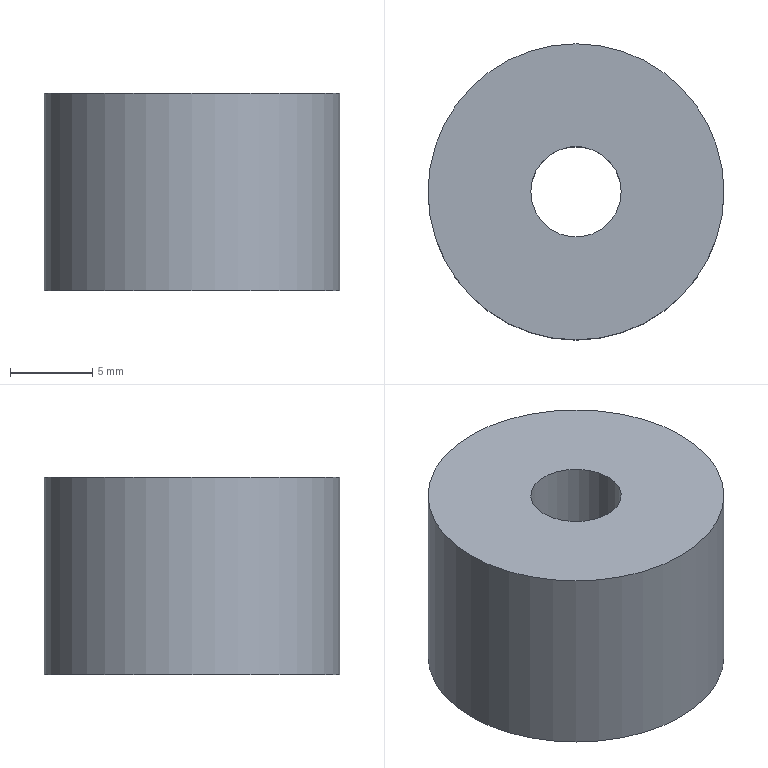Component | NX | BASE_LOC_BLOCK | 1 solid | 6 faces | box 18 x 18 x 12 mm | volume 2473 mm3 | plane 3 | cylinder 3 | commonest cylinder face diameters 18 x1 5.5 x1 10 x1
STEP:
#1=CARTESIAN_POINT('',(0.,0.,0.));
#2=DIRECTION('',(0.,0.,1.));
#3=DIRECTION('',(1.,0.,0.));
#4=AXIS2_PLACEMENT_3D('',#1,#2,#3);
#5=CARTESIAN_POINT('',(110.,0.,-272.));
#6=VERTEX_POINT('',#5);
#7=CARTESIAN_POINT('',(115.,0.,-272.));
#8=DIRECTION('',(0.,0.,1.));
#9=DIRECTION('',(-1.,0.,0.));
#10=AXIS2_PLACEMENT_3D('',#7,#8,#9);
#11=CIRCLE('',#10,5.);
#12=CARTESIAN_POINT('',(115.,0.,-272.));
#13=DIRECTION('',(0.,0.,-1.));
#14=DIRECTION('',(1.,0.,0.));
#15=AXIS2_PLACEMENT_3D('',#12,#13,#14);
#16=PLANE('',#15);
#17=CARTESIAN_POINT('',(-5.,0.));
#18=CARTESIAN_POINT('',(-5.,8.66));
#19=CARTESIAN_POINT('',(2.5,4.33));
#20=CARTESIAN_POINT('',(10.,0.));
#21=CARTESIAN_POINT('',(2.5,-4.33));
#22=CARTESIAN_POINT('',(-5.,-8.66));
#23=CARTESIAN_POINT('',(-5.,0.));
#24=(BOUNDED_CURVE()B_SPLINE_CURVE(2,(#17,#18,#19,#20,#21,#22,#23),.UNSPECIFIED.,.T.,.F.)B_SPLINE_CURVE_WITH_KNOTS((1,2,2,2,2,1),(-2.094,0.,2.094,4.189,6.283,8.378),.UNSPECIFIED.)CURVE()GEOMETRIC_REPRESENTATION_ITEM()RATIONAL_B_SPLINE_CURVE((1.,0.5,1.,0.5,1.,0.5,1.))REPRESENTATION_ITEM(''));
#25=(GEOMETRIC_REPRESENTATION_CONTEXT(2)PARAMETRIC_REPRESENTATION_CONTEXT()REPRESENTATION_CONTEXT('',''));
#26=DEFINITIONAL_REPRESENTATION('',(#24),#25);
#27=PCURVE('',#16,#26);
#28=CARTESIAN_POINT('',(115.,0.,-272.));
#29=DIRECTION('',(0.,0.,1.));
#30=DIRECTION('',(-1.,0.,0.));
#31=AXIS2_PLACEMENT_3D('',#28,#29,#30);
#32=CYLINDRICAL_SURFACE('',#31,5.);
#33=CARTESIAN_POINT('',(0.,0.));
#34=DIRECTION('',(1.,0.));
#35=VECTOR('',#34,1.);
#36=LINE('',#33,#35);
#37=(GEOMETRIC_REPRESENTATION_CONTEXT(2)PARAMETRIC_REPRESENTATION_CONTEXT()REPRESENTATION_CONTEXT('',''));
#38=DEFINITIONAL_REPRESENTATION('',(#36),#37);
#39=PCURVE('',#32,#38);
#40=SURFACE_CURVE('',#11,(#27,#39),.PCURVE_S1.);
#41=EDGE_CURVE('',#6,#6,#40,.T.);
#42=ORIENTED_EDGE('',*,*,#41,.T.);
#43=EDGE_LOOP('',(#42));
#44=FACE_BOUND('',#43,.T.);
#45=CARTESIAN_POINT('',(124.,0.,-272.));
#46=VERTEX_POINT('',#45);
#47=CARTESIAN_POINT('',(115.,0.,-272.));
#48=DIRECTION('',(0.,0.,1.));
#49=DIRECTION('',(1.,0.,0.));
#50=AXIS2_PLACEMENT_3D('',#47,#48,#49);
#51=CIRCLE('',#50,9.);
#52=CARTESIAN_POINT('',(9.,0.));
#53=CARTESIAN_POINT('',(9.,-15.588));
#54=CARTESIAN_POINT('',(-4.5,-7.794));
#55=CARTESIAN_POINT('',(-18.,-0.));
#56=CARTESIAN_POINT('',(-4.5,7.794));
#57=CARTESIAN_POINT('',(9.,15.588));
#58=CARTESIAN_POINT('',(9.,0.));
#59=(BOUNDED_CURVE()B_SPLINE_CURVE(2,(#52,#53,#54,#55,#56,#57,#58),.UNSPECIFIED.,.T.,.F.)B_SPLINE_CURVE_WITH_KNOTS((1,2,2,2,2,1),(-2.094,0.,2.094,4.189,6.283,8.378),.UNSPECIFIED.)CURVE()GEOMETRIC_REPRESENTATION_ITEM()RATIONAL_B_SPLINE_CURVE((1.,0.5,1.,0.5,1.,0.5,1.))REPRESENTATION_ITEM(''));
#60=(GEOMETRIC_REPRESENTATION_CONTEXT(2)PARAMETRIC_REPRESENTATION_CONTEXT()REPRESENTATION_CONTEXT('',''));
#61=DEFINITIONAL_REPRESENTATION('',(#59),#60);
#62=PCURVE('',#16,#61);
#63=CARTESIAN_POINT('',(115.,0.,-260.));
#64=DIRECTION('',(0.,0.,-1.));
#65=DIRECTION('',(1.,0.,0.));
#66=AXIS2_PLACEMENT_3D('',#63,#64,#65);
#67=CYLINDRICAL_SURFACE('',#66,9.);
#68=CARTESIAN_POINT('',(6.283,12.));
#69=DIRECTION('',(-1.,0.));
#70=VECTOR('',#69,1.);
#71=LINE('',#68,#70);
#72=(GEOMETRIC_REPRESENTATION_CONTEXT(2)PARAMETRIC_REPRESENTATION_CONTEXT()REPRESENTATION_CONTEXT('',''));
#73=DEFINITIONAL_REPRESENTATION('',(#71),#72);
#74=PCURVE('',#67,#73);
#75=SURFACE_CURVE('',#51,(#62,#74),.PCURVE_S1.);
#76=EDGE_CURVE('',#46,#46,#75,.T.);
#77=ORIENTED_EDGE('',*,*,#76,.F.);
#78=EDGE_LOOP('',(#77));
#79=FACE_BOUND('',#78,.T.);
#80=ADVANCED_FACE('',(#44,#79),#16,.T.);
#81=CARTESIAN_POINT('',(112.25,0.,-260.));
#82=VERTEX_POINT('',#81);
#83=CARTESIAN_POINT('',(115.,0.,-260.));
#84=DIRECTION('',(0.,0.,1.));
#85=DIRECTION('',(-1.,0.,0.));
#86=AXIS2_PLACEMENT_3D('',#83,#84,#85);
#87=CIRCLE('',#86,2.75);
#88=CARTESIAN_POINT('',(115.,0.,-260.));
#89=DIRECTION('',(0.,0.,1.));
#90=DIRECTION('',(-1.,0.,0.));
#91=AXIS2_PLACEMENT_3D('',#88,#89,#90);
#92=PLANE('',#91);
#93=CARTESIAN_POINT('',(0.,0.));
#94=DIRECTION('',(1.,0.));
#95=AXIS2_PLACEMENT_2D('',#93,#94);
#96=CIRCLE('',#95,2.75);
#97=(GEOMETRIC_REPRESENTATION_CONTEXT(2)PARAMETRIC_REPRESENTATION_CONTEXT()REPRESENTATION_CONTEXT('',''));
#98=DEFINITIONAL_REPRESENTATION('',(#96),#97);
#99=PCURVE('',#92,#98);
#100=CARTESIAN_POINT('',(115.,0.,-222.));
#101=DIRECTION('',(0.,0.,1.));
#102=DIRECTION('',(-1.,0.,0.));
#103=AXIS2_PLACEMENT_3D('',#100,#101,#102);
#104=CYLINDRICAL_SURFACE('',#103,2.75);
#105=CARTESIAN_POINT('',(0.,-38.));
#106=DIRECTION('',(1.,0.));
#107=VECTOR('',#106,1.);
#108=LINE('',#105,#107);
#109=(GEOMETRIC_REPRESENTATION_CONTEXT(2)PARAMETRIC_REPRESENTATION_CONTEXT()REPRESENTATION_CONTEXT('',''));
#110=DEFINITIONAL_REPRESENTATION('',(#108),#109);
#111=PCURVE('',#104,#110);
#112=SURFACE_CURVE('',#87,(#99,#111),.PCURVE_S1.);
#113=EDGE_CURVE('',#82,#82,#112,.T.);
#114=ORIENTED_EDGE('',*,*,#113,.F.);
#115=EDGE_LOOP('',(#114));
#116=FACE_BOUND('',#115,.T.);
#117=CARTESIAN_POINT('',(124.,0.,-260.));
#118=VERTEX_POINT('',#117);
#119=CARTESIAN_POINT('',(115.,0.,-260.));
#120=DIRECTION('',(0.,0.,-1.));
#121=DIRECTION('',(1.,0.,0.));
#122=AXIS2_PLACEMENT_3D('',#119,#120,#121);
#123=CIRCLE('',#122,9.);
#124=CARTESIAN_POINT('',(-9.,0.));
#125=CARTESIAN_POINT('',(-9.,15.588));
#126=CARTESIAN_POINT('',(4.5,7.794));
#127=CARTESIAN_POINT('',(18.,0.));
#128=CARTESIAN_POINT('',(4.5,-7.794));
#129=CARTESIAN_POINT('',(-9.,-15.588));
#130=CARTESIAN_POINT('',(-9.,0.));
#131=(BOUNDED_CURVE()B_SPLINE_CURVE(2,(#124,#125,#126,#127,#128,#129,#130),.UNSPECIFIED.,.T.,.F.)B_SPLINE_CURVE_WITH_KNOTS((1,2,2,2,2,1),(-2.094,0.,2.094,4.189,6.283,8.378),.UNSPECIFIED.)CURVE()GEOMETRIC_REPRESENTATION_ITEM()RATIONAL_B_SPLINE_CURVE((1.,0.5,1.,0.5,1.,0.5,1.))REPRESENTATION_ITEM(''));
#132=(GEOMETRIC_REPRESENTATION_CONTEXT(2)PARAMETRIC_REPRESENTATION_CONTEXT()REPRESENTATION_CONTEXT('',''));
#133=DEFINITIONAL_REPRESENTATION('',(#131),#132);
#134=PCURVE('',#92,#133);
#135=CARTESIAN_POINT('',(0.,0.));
#136=DIRECTION('',(1.,0.));
#137=VECTOR('',#136,1.);
#138=LINE('',#135,#137);
#139=(GEOMETRIC_REPRESENTATION_CONTEXT(2)PARAMETRIC_REPRESENTATION_CONTEXT()REPRESENTATION_CONTEXT('',''));
#140=DEFINITIONAL_REPRESENTATION('',(#138),#139);
#141=PCURVE('',#67,#140);
#142=SURFACE_CURVE('',#123,(#134,#141),.PCURVE_S1.);
#143=EDGE_CURVE('',#118,#118,#142,.T.);
#144=ORIENTED_EDGE('',*,*,#143,.F.);
#145=EDGE_LOOP('',(#144));
#146=FACE_BOUND('',#145,.T.);
#147=ADVANCED_FACE('',(#116,#146),#92,.T.);
#148=ORIENTED_EDGE('',*,*,#76,.T.);
#149=CARTESIAN_POINT('',(124.,0.,-260.));
#150=CARTESIAN_POINT('',(124.,0.,-272.));
#151=B_SPLINE_CURVE_WITH_KNOTS('',1,(#149,#150),.UNSPECIFIED.,.F.,.F.,(2,2),(0.,12.),.PIECEWISE_BEZIER_KNOTS.);
#152=CARTESIAN_POINT('',(0.,0.));
#153=DIRECTION('',(0.,1.));
#154=VECTOR('',#153,1.);
#155=LINE('',#152,#154);
#156=(GEOMETRIC_REPRESENTATION_CONTEXT(2)PARAMETRIC_REPRESENTATION_CONTEXT()REPRESENTATION_CONTEXT('',''));
#157=DEFINITIONAL_REPRESENTATION('',(#155),#156);
#158=PCURVE('',#67,#157);
#159=CARTESIAN_POINT('',(6.283,0.));
#160=DIRECTION('',(0.,1.));
#161=VECTOR('',#160,1.);
#162=LINE('',#159,#161);
#163=(GEOMETRIC_REPRESENTATION_CONTEXT(2)PARAMETRIC_REPRESENTATION_CONTEXT()REPRESENTATION_CONTEXT('',''));
#164=DEFINITIONAL_REPRESENTATION('',(#162),#163);
#165=PCURVE('',#67,#164);
#166=SEAM_CURVE('',#151,(#158,#165),.PCURVE_S1.);
#167=EDGE_CURVE('',#118,#46,#166,.T.);
#168=ORIENTED_EDGE('',*,*,#167,.F.);
#169=ORIENTED_EDGE('',*,*,#143,.T.);
#170=ORIENTED_EDGE('',*,*,#167,.T.);
#171=EDGE_LOOP('',(#148,#168,#169,#170));
#172=FACE_BOUND('',#171,.T.);
#173=ADVANCED_FACE('',(#172),#67,.T.);
#174=ORIENTED_EDGE('',*,*,#113,.F.);
#175=CARTESIAN_POINT('',(112.25,0.,-266.6));
#176=VERTEX_POINT('',#175);
#177=CARTESIAN_POINT('',(112.25,0.,-266.6));
#178=CARTESIAN_POINT('',(112.25,0.,-260.));
#179=B_SPLINE_CURVE_WITH_KNOTS('',1,(#177,#178),.UNSPECIFIED.,.F.,.F.,(2,2),(-44.6,-38.),.PIECEWISE_BEZIER_KNOTS.);
#180=CARTESIAN_POINT('',(0.,0.));
#181=DIRECTION('',(0.,1.));
#182=VECTOR('',#181,1.);
#183=LINE('',#180,#182);
#184=(GEOMETRIC_REPRESENTATION_CONTEXT(2)PARAMETRIC_REPRESENTATION_CONTEXT()REPRESENTATION_CONTEXT('',''));
#185=DEFINITIONAL_REPRESENTATION('',(#183),#184);
#186=PCURVE('',#104,#185);
#187=CARTESIAN_POINT('',(6.283,0.));
#188=DIRECTION('',(0.,1.));
#189=VECTOR('',#188,1.);
#190=LINE('',#187,#189);
#191=(GEOMETRIC_REPRESENTATION_CONTEXT(2)PARAMETRIC_REPRESENTATION_CONTEXT()REPRESENTATION_CONTEXT('',''));
#192=DEFINITIONAL_REPRESENTATION('',(#190),#191);
#193=PCURVE('',#104,#192);
#194=SEAM_CURVE('',#179,(#186,#193),.PCURVE_S1.);
#195=EDGE_CURVE('',#176,#82,#194,.T.);
#196=ORIENTED_EDGE('',*,*,#195,.F.);
#197=CARTESIAN_POINT('',(115.,0.,-266.6));
#198=DIRECTION('',(0.,0.,-1.));
#199=DIRECTION('',(-1.,0.,0.));
#200=AXIS2_PLACEMENT_3D('',#197,#198,#199);
#201=CIRCLE('',#200,2.75);
#202=CARTESIAN_POINT('',(6.283,-44.6));
#203=DIRECTION('',(-1.,0.));
#204=VECTOR('',#203,1.);
#205=LINE('',#202,#204);
#206=(GEOMETRIC_REPRESENTATION_CONTEXT(2)PARAMETRIC_REPRESENTATION_CONTEXT()REPRESENTATION_CONTEXT('',''));
#207=DEFINITIONAL_REPRESENTATION('',(#205),#206);
#208=PCURVE('',#104,#207);
#209=CARTESIAN_POINT('',(115.,0.,-266.6));
#210=DIRECTION('',(0.,0.,1.));
#211=DIRECTION('',(-1.,0.,0.));
#212=AXIS2_PLACEMENT_3D('',#209,#210,#211);
#213=PLANE('',#212);
#214=CARTESIAN_POINT('',(2.75,0.));
#215=CARTESIAN_POINT('',(2.75,-4.763));
#216=CARTESIAN_POINT('',(-1.375,-2.382));
#217=CARTESIAN_POINT('',(-5.5,-0.));
#218=CARTESIAN_POINT('',(-1.375,2.382));
#219=CARTESIAN_POINT('',(2.75,4.763));
#220=CARTESIAN_POINT('',(2.75,0.));
#221=(BOUNDED_CURVE()B_SPLINE_CURVE(2,(#214,#215,#216,#217,#218,#219,#220),.UNSPECIFIED.,.T.,.F.)B_SPLINE_CURVE_WITH_KNOTS((1,2,2,2,2,1),(-2.094,0.,2.094,4.189,6.283,8.378),.UNSPECIFIED.)CURVE()GEOMETRIC_REPRESENTATION_ITEM()RATIONAL_B_SPLINE_CURVE((1.,0.5,1.,0.5,1.,0.5,1.))REPRESENTATION_ITEM(''));
#222=(GEOMETRIC_REPRESENTATION_CONTEXT(2)PARAMETRIC_REPRESENTATION_CONTEXT()REPRESENTATION_CONTEXT('',''));
#223=DEFINITIONAL_REPRESENTATION('',(#221),#222);
#224=PCURVE('',#213,#223);
#225=SURFACE_CURVE('',#201,(#208,#224),.PCURVE_S1.);
#226=EDGE_CURVE('',#176,#176,#225,.T.);
#227=ORIENTED_EDGE('',*,*,#226,.F.);
#228=ORIENTED_EDGE('',*,*,#195,.T.);
#229=EDGE_LOOP('',(#174,#196,#227,#228));
#230=FACE_BOUND('',#229,.F.);
#231=ADVANCED_FACE('',(#230),#104,.F.);
#232=ORIENTED_EDGE('',*,*,#226,.F.);
#233=EDGE_LOOP('',(#232));
#234=FACE_BOUND('',#233,.T.);
#235=CARTESIAN_POINT('',(110.,0.,-266.6));
#236=VERTEX_POINT('',#235);
#237=CARTESIAN_POINT('',(115.,0.,-266.6));
#238=DIRECTION('',(0.,0.,-1.));
#239=DIRECTION('',(-1.,0.,0.));
#240=AXIS2_PLACEMENT_3D('',#237,#238,#239);
#241=CIRCLE('',#240,5.);
#242=CARTESIAN_POINT('',(5.,0.));
#243=CARTESIAN_POINT('',(5.,-8.66));
#244=CARTESIAN_POINT('',(-2.5,-4.33));
#245=CARTESIAN_POINT('',(-10.,-0.));
#246=CARTESIAN_POINT('',(-2.5,4.33));
#247=CARTESIAN_POINT('',(5.,8.66));
#248=CARTESIAN_POINT('',(5.,0.));
#249=(BOUNDED_CURVE()B_SPLINE_CURVE(2,(#242,#243,#244,#245,#246,#247,#248),.UNSPECIFIED.,.T.,.F.)B_SPLINE_CURVE_WITH_KNOTS((1,2,2,2,2,1),(-2.094,0.,2.094,4.189,6.283,8.378),.UNSPECIFIED.)CURVE()GEOMETRIC_REPRESENTATION_ITEM()RATIONAL_B_SPLINE_CURVE((1.,0.5,1.,0.5,1.,0.5,1.))REPRESENTATION_ITEM(''));
#250=(GEOMETRIC_REPRESENTATION_CONTEXT(2)PARAMETRIC_REPRESENTATION_CONTEXT()REPRESENTATION_CONTEXT('',''));
#251=DEFINITIONAL_REPRESENTATION('',(#249),#250);
#252=PCURVE('',#213,#251);
#253=CARTESIAN_POINT('',(6.283,5.4));
#254=DIRECTION('',(-1.,0.));
#255=VECTOR('',#254,1.);
#256=LINE('',#253,#255);
#257=(GEOMETRIC_REPRESENTATION_CONTEXT(2)PARAMETRIC_REPRESENTATION_CONTEXT()REPRESENTATION_CONTEXT('',''));
#258=DEFINITIONAL_REPRESENTATION('',(#256),#257);
#259=PCURVE('',#32,#258);
#260=SURFACE_CURVE('',#241,(#252,#259),.PCURVE_S1.);
#261=EDGE_CURVE('',#236,#236,#260,.T.);
#262=ORIENTED_EDGE('',*,*,#261,.T.);
#263=EDGE_LOOP('',(#262));
#264=FACE_BOUND('',#263,.T.);
#265=ADVANCED_FACE('',(#234,#264),#213,.F.);
#266=ORIENTED_EDGE('',*,*,#261,.T.);
#267=CARTESIAN_POINT('',(110.,0.,-272.));
#268=CARTESIAN_POINT('',(110.,0.,-266.6));
#269=B_SPLINE_CURVE_WITH_KNOTS('',1,(#267,#268),.UNSPECIFIED.,.F.,.F.,(2,2),(0.,5.4),.PIECEWISE_BEZIER_KNOTS.);
#270=CARTESIAN_POINT('',(0.,0.));
#271=DIRECTION('',(0.,1.));
#272=VECTOR('',#271,1.);
#273=LINE('',#270,#272);
#274=(GEOMETRIC_REPRESENTATION_CONTEXT(2)PARAMETRIC_REPRESENTATION_CONTEXT()REPRESENTATION_CONTEXT('',''));
#275=DEFINITIONAL_REPRESENTATION('',(#273),#274);
#276=PCURVE('',#32,#275);
#277=CARTESIAN_POINT('',(6.283,0.));
#278=DIRECTION('',(0.,1.));
#279=VECTOR('',#278,1.);
#280=LINE('',#277,#279);
#281=(GEOMETRIC_REPRESENTATION_CONTEXT(2)PARAMETRIC_REPRESENTATION_CONTEXT()REPRESENTATION_CONTEXT('',''));
#282=DEFINITIONAL_REPRESENTATION('',(#280),#281);
#283=PCURVE('',#32,#282);
#284=SEAM_CURVE('',#269,(#276,#283),.PCURVE_S1.);
#285=EDGE_CURVE('',#6,#236,#284,.T.);
#286=ORIENTED_EDGE('',*,*,#285,.F.);
#287=ORIENTED_EDGE('',*,*,#41,.T.);
#288=ORIENTED_EDGE('',*,*,#285,.T.);
#289=EDGE_LOOP('',(#266,#286,#287,#288));
#290=FACE_BOUND('',#289,.F.);
#291=ADVANCED_FACE('',(#290),#32,.F.);
#292=CLOSED_SHELL('',(#80,#147,#173,#231,#265,#291));
#293=MANIFOLD_SOLID_BREP('',#292);
#294=(LENGTH_UNIT()NAMED_UNIT(*)SI_UNIT(.MILLI.,.METRE.));
#295=UNCERTAINTY_MEASURE_WITH_UNIT(LENGTH_MEASURE(0.00001),#294,'','');
#296=(NAMED_UNIT(*)PLANE_ANGLE_UNIT()SI_UNIT($,.RADIAN.));
#297=(NAMED_UNIT(*)SI_UNIT($,.STERADIAN.)SOLID_ANGLE_UNIT());
#298=(GEOMETRIC_REPRESENTATION_CONTEXT(3)GLOBAL_UNCERTAINTY_ASSIGNED_CONTEXT((#295))GLOBAL_UNIT_ASSIGNED_CONTEXT((#294,#296,#297))REPRESENTATION_CONTEXT('',''));
#299=ADVANCED_BREP_SHAPE_REPRESENTATION('',(#4,#293),#298);